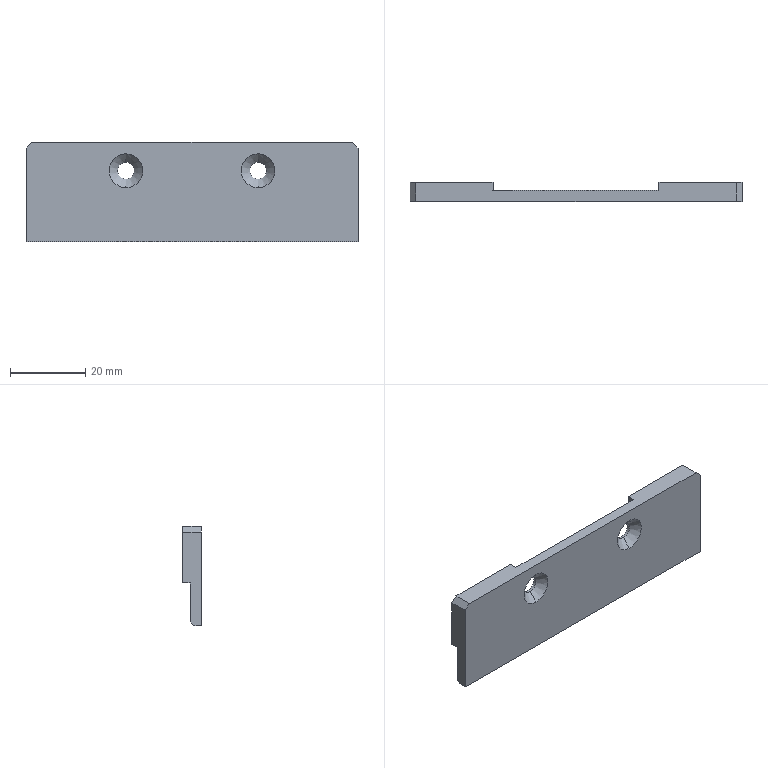Component | SolidWorks | 12-DividingMechanism-1111-1_17-1111-2 | 1 solid | 23 faces | box 88 x 5 x 26.3 mm | volume 8019 mm3 | plane 15 | cone 4 | cylinder 4 | commonest cylinder face diameters 4.5 x4
build123d program:
from build123d import *

# Parameters (mm, degrees)
SKETCH5_W                                            = 88
SKETCH5_H                                            = 26.3
BOSS_EXTRUDE1_DEPTH                                  = 5
SKETCH6_W                                            = 44
SKETCH6_H                                            = 26.3
CUT_EXTRUDE1_DEPTH                                   = 2
SKETCH7_W                                            = 88
SKETCH7_H                                            = 11.3
CUT_EXTRUDE2_DEPTH                                   = 2
CHAMFER1_SIZE                                        = 1
CHAMFER2_SIZE                                        = 1.5
M4_HEXAGON_SOCKET_COUNTERSUNK_HEAD_SCREW_D           = 4.5
M4_HEXAGON_SOCKET_COUNTERSUNK_HEAD_SCREW_CSINK_D     = 8.96
M4_HEXAGON_SOCKET_COUNTERSUNK_HEAD_SCREW_CSINK_ANGLE = 90


with BuildPart() as part:
    # Sketch5 → Boss-Extrude1 (new body)
    with BuildSketch(Plane(origin=(0, 0, 0), x_dir=(1, 0, 0), z_dir=(0, 1, 0))):
        Rectangle(SKETCH5_W, SKETCH5_H)
    extrude(amount=BOSS_EXTRUDE1_DEPTH)

    # Sketch6 → Cut-Extrude1 (cut)
    with BuildSketch(Plane(origin=(0, 5, 0), x_dir=(1, 0, 0), z_dir=(0, 1, 0))):
        Rectangle(SKETCH6_W, SKETCH6_H)
    extrude(amount=-CUT_EXTRUDE1_DEPTH, mode=Mode.SUBTRACT)

    # Sketch7 → Cut-Extrude2 (cut)
    with BuildSketch(Plane(origin=(0, 5, 0), x_dir=(1, 0, 0), z_dir=(0, 1, 0))):
        with Locations((0, -7.5)):
            Rectangle(SKETCH7_W, SKETCH7_H)
    extrude(amount=-CUT_EXTRUDE2_DEPTH, mode=Mode.SUBTRACT)

    # Chamfer1
    chamfer1_edges = [part.edges().sort_by_distance(p)[0] for p in [
        (0, 3, 13.15),
    ]]
    chamfer(chamfer1_edges, length=CHAMFER1_SIZE)

    # Chamfer2
    chamfer2_edges = [part.edges().sort_by_distance(p)[0] for p in [
        (-44, 2.5, -13.15),
        (44, 2.5, -13.15),
    ]]
    chamfer(chamfer2_edges, length=CHAMFER2_SIZE)

    # M4 Hexagon Socket Countersunk Head Screw (through all)
    with Locations(Plane(origin=(0, 0, 0), x_dir=(-1, 0, 0), z_dir=(0, -1, 0))):
        with Locations((-17.5, 5.65), (17.5, 5.65)):
            CounterSinkHole(M4_HEXAGON_SOCKET_COUNTERSUNK_HEAD_SCREW_D / 2, M4_HEXAGON_SOCKET_COUNTERSUNK_HEAD_SCREW_CSINK_D / 2, counter_sink_angle=M4_HEXAGON_SOCKET_COUNTERSUNK_HEAD_SCREW_CSINK_ANGLE)


solid = part.part

# Placed as in the assembly
solid = solid.moved(Location((3.428, 571.024, 1511.906), (-180, 0, 180)))
STEP:
#1=COLOUR_RGB('',0.7922,0.8196,0.9333);
#2=FILL_AREA_STYLE_COLOUR('',#1);
#3=FILL_AREA_STYLE('',(#2));
#4=SURFACE_STYLE_FILL_AREA(#3);
#5=SURFACE_SIDE_STYLE('',(#4));
#6=SURFACE_STYLE_USAGE(.BOTH.,#5);
#7=PRESENTATION_STYLE_ASSIGNMENT((#6));
#8=CARTESIAN_POINT('',(-0.554,22.569,59.658));
#9=VERTEX_POINT('',#8);
#10=CARTESIAN_POINT('',(-0.554,22.569,59.835));
#11=VERTEX_POINT('',#10);
#12=CARTESIAN_POINT('',(-0.554,22.569,59.746));
#13=DIRECTION('',(-0.,-1.,0.));
#14=DIRECTION('',(0.,0.,1.));
#15=AXIS2_PLACEMENT_3D('',#12,#13,#14);
#16=CIRCLE('',#15,0.08858);
#17=EDGE_CURVE('',#9,#11,#16,.T.);
#18=ORIENTED_EDGE('',*,*,#17,.F.);
#19=CARTESIAN_POINT('',(-0.554,22.481,59.57));
#20=VERTEX_POINT('',#19);
#21=CARTESIAN_POINT('',(-0.554,22.481,59.57));
#22=DIRECTION('',(-0.,-0.7071,-0.7071));
#23=VECTOR('',#22,39.37);
#24=LINE('',#21,#23);
#25=EDGE_CURVE('',#9,#20,#24,.T.);
#26=ORIENTED_EDGE('',*,*,#25,.T.);
#27=CARTESIAN_POINT('',(-0.554,22.481,59.923));
#28=VERTEX_POINT('',#27);
#29=CARTESIAN_POINT('',(-0.554,22.481,59.746));
#30=DIRECTION('',(-0.,-1.,0.));
#31=DIRECTION('',(0.,0.,1.));
#32=AXIS2_PLACEMENT_3D('',#29,#30,#31);
#33=CIRCLE('',#32,0.1764);
#34=EDGE_CURVE('',#20,#28,#33,.T.);
#35=ORIENTED_EDGE('',*,*,#34,.T.);
#36=CARTESIAN_POINT('',(-0.554,22.481,59.923));
#37=DIRECTION('',(-0.,-0.7071,0.7071));
#38=VECTOR('',#37,39.37);
#39=LINE('',#36,#38);
#40=EDGE_CURVE('',#11,#28,#39,.T.);
#41=ORIENTED_EDGE('',*,*,#40,.F.);
#42=EDGE_LOOP('',(#18,#26,#35,#41));
#43=FACE_OUTER_BOUND('',#42,.T.);
#44=CARTESIAN_POINT('',(-0.554,22.481,59.746));
#45=DIRECTION('',(-0.,-1.,0.));
#46=DIRECTION('',(0.,0.,1.));
#47=AXIS2_PLACEMENT_3D('',#44,#45,#46);
#48=CONICAL_SURFACE('',#47,0.1764,0.7854);
#49=ADVANCED_FACE('',(#43),#48,.F.);
#50=CARTESIAN_POINT('',(-0.554,22.599,59.658));
#51=VERTEX_POINT('',#50);
#52=CARTESIAN_POINT('',(-0.554,22.599,59.835));
#53=VERTEX_POINT('',#52);
#54=CARTESIAN_POINT('',(-0.554,22.599,59.746));
#55=DIRECTION('',(-0.,-1.,0.));
#56=DIRECTION('',(0.,0.,1.));
#57=AXIS2_PLACEMENT_3D('',#54,#55,#56);
#58=CIRCLE('',#57,0.08858);
#59=EDGE_CURVE('',#51,#53,#58,.T.);
#60=ORIENTED_EDGE('',*,*,#59,.F.);
#61=CARTESIAN_POINT('',(-0.554,22.481,59.658));
#62=DIRECTION('',(-0.,-1.,0.));
#63=VECTOR('',#62,39.37);
#64=LINE('',#61,#63);
#65=EDGE_CURVE('',#51,#9,#64,.T.);
#66=ORIENTED_EDGE('',*,*,#65,.T.);
#67=ORIENTED_EDGE('',*,*,#17,.T.);
#68=CARTESIAN_POINT('',(-0.554,22.481,59.835));
#69=DIRECTION('',(-0.,-1.,0.));
#70=VECTOR('',#69,39.37);
#71=LINE('',#68,#70);
#72=EDGE_CURVE('',#53,#11,#71,.T.);
#73=ORIENTED_EDGE('',*,*,#72,.F.);
#74=EDGE_LOOP('',(#60,#66,#67,#73));
#75=FACE_OUTER_BOUND('',#74,.T.);
#76=CARTESIAN_POINT('',(-0.554,22.481,59.746));
#77=DIRECTION('',(-0.,-1.,0.));
#78=DIRECTION('',(0.,0.,1.));
#79=AXIS2_PLACEMENT_3D('',#76,#77,#78);
#80=CYLINDRICAL_SURFACE('',#79,0.08858);
#81=ADVANCED_FACE('',(#75),#80,.F.);
#82=CARTESIAN_POINT('',(0.8239,22.569,59.658));
#83=VERTEX_POINT('',#82);
#84=CARTESIAN_POINT('',(0.8239,22.569,59.835));
#85=VERTEX_POINT('',#84);
#86=CARTESIAN_POINT('',(0.8239,22.569,59.746));
#87=DIRECTION('',(-0.,-1.,0.));
#88=DIRECTION('',(0.,0.,1.));
#89=AXIS2_PLACEMENT_3D('',#86,#87,#88);
#90=CIRCLE('',#89,0.08858);
#91=EDGE_CURVE('',#83,#85,#90,.T.);
#92=ORIENTED_EDGE('',*,*,#91,.F.);
#93=CARTESIAN_POINT('',(0.8239,22.481,59.57));
#94=VERTEX_POINT('',#93);
#95=CARTESIAN_POINT('',(0.8239,22.481,59.57));
#96=DIRECTION('',(-0.,-0.7071,-0.7071));
#97=VECTOR('',#96,39.37);
#98=LINE('',#95,#97);
#99=EDGE_CURVE('',#83,#94,#98,.T.);
#100=ORIENTED_EDGE('',*,*,#99,.T.);
#101=CARTESIAN_POINT('',(0.8239,22.481,59.923));
#102=VERTEX_POINT('',#101);
#103=CARTESIAN_POINT('',(0.8239,22.481,59.746));
#104=DIRECTION('',(-0.,-1.,0.));
#105=DIRECTION('',(0.,0.,1.));
#106=AXIS2_PLACEMENT_3D('',#103,#104,#105);
#107=CIRCLE('',#106,0.1764);
#108=EDGE_CURVE('',#94,#102,#107,.T.);
#109=ORIENTED_EDGE('',*,*,#108,.T.);
#110=CARTESIAN_POINT('',(0.8239,22.481,59.923));
#111=DIRECTION('',(-0.,-0.7071,0.7071));
#112=VECTOR('',#111,39.37);
#113=LINE('',#110,#112);
#114=EDGE_CURVE('',#85,#102,#113,.T.);
#115=ORIENTED_EDGE('',*,*,#114,.F.);
#116=EDGE_LOOP('',(#92,#100,#109,#115));
#117=FACE_OUTER_BOUND('',#116,.T.);
#118=CARTESIAN_POINT('',(0.8239,22.481,59.746));
#119=DIRECTION('',(-0.,-1.,0.));
#120=DIRECTION('',(0.,0.,1.));
#121=AXIS2_PLACEMENT_3D('',#118,#119,#120);
#122=CONICAL_SURFACE('',#121,0.1764,0.7854);
#123=ADVANCED_FACE('',(#117),#122,.F.);
#124=CARTESIAN_POINT('',(0.8239,22.599,59.658));
#125=VERTEX_POINT('',#124);
#126=CARTESIAN_POINT('',(0.8239,22.599,59.835));
#127=VERTEX_POINT('',#126);
#128=CARTESIAN_POINT('',(0.8239,22.599,59.746));
#129=DIRECTION('',(-0.,-1.,0.));
#130=DIRECTION('',(0.,0.,1.));
#131=AXIS2_PLACEMENT_3D('',#128,#129,#130);
#132=CIRCLE('',#131,0.08858);
#133=EDGE_CURVE('',#125,#127,#132,.T.);
#134=ORIENTED_EDGE('',*,*,#133,.F.);
#135=CARTESIAN_POINT('',(0.8239,22.481,59.658));
#136=DIRECTION('',(-0.,-1.,0.));
#137=VECTOR('',#136,39.37);
#138=LINE('',#135,#137);
#139=EDGE_CURVE('',#125,#83,#138,.T.);
#140=ORIENTED_EDGE('',*,*,#139,.T.);
#141=ORIENTED_EDGE('',*,*,#91,.T.);
#142=CARTESIAN_POINT('',(0.8239,22.481,59.835));
#143=DIRECTION('',(-0.,-1.,0.));
#144=VECTOR('',#143,39.37);
#145=LINE('',#142,#144);
#146=EDGE_CURVE('',#127,#85,#145,.T.);
#147=ORIENTED_EDGE('',*,*,#146,.F.);
#148=EDGE_LOOP('',(#134,#140,#141,#147));
#149=FACE_OUTER_BOUND('',#148,.T.);
#150=CARTESIAN_POINT('',(0.8239,22.481,59.746));
#151=DIRECTION('',(-0.,-1.,0.));
#152=DIRECTION('',(0.,0.,1.));
#153=AXIS2_PLACEMENT_3D('',#150,#151,#152);
#154=CYLINDRICAL_SURFACE('',#153,0.08858);
#155=ADVANCED_FACE('',(#149),#154,.F.);
#156=CARTESIAN_POINT('',(-1.597,22.678,59.451));
#157=VERTEX_POINT('',#156);
#158=CARTESIAN_POINT('',(-1.597,22.678,59.983));
#159=VERTEX_POINT('',#158);
#160=CARTESIAN_POINT('',(-1.597,22.678,59.006));
#161=DIRECTION('',(-0.,0.,1.));
#162=VECTOR('',#161,39.37);
#163=LINE('',#160,#162);
#164=EDGE_CURVE('',#157,#159,#163,.T.);
#165=ORIENTED_EDGE('',*,*,#164,.T.);
#166=CARTESIAN_POINT('',(-1.538,22.678,60.042));
#167=VERTEX_POINT('',#166);
#168=CARTESIAN_POINT('',(-0.9605,22.678,60.619));
#169=DIRECTION('',(0.7071,0.,0.7071));
#170=VECTOR('',#169,39.37);
#171=LINE('',#168,#170);
#172=EDGE_CURVE('',#159,#167,#171,.T.);
#173=ORIENTED_EDGE('',*,*,#172,.T.);
#174=CARTESIAN_POINT('',(-0.7312,22.678,60.042));
#175=VERTEX_POINT('',#174);
#176=CARTESIAN_POINT('',(-1.597,22.678,60.042));
#177=DIRECTION('',(1.,-0.,-0.));
#178=VECTOR('',#177,39.37);
#179=LINE('',#176,#178);
#180=EDGE_CURVE('',#167,#175,#179,.T.);
#181=ORIENTED_EDGE('',*,*,#180,.T.);
#182=CARTESIAN_POINT('',(-0.7312,22.678,59.451));
#183=VERTEX_POINT('',#182);
#184=CARTESIAN_POINT('',(-0.7312,22.678,59.006));
#185=DIRECTION('',(-0.,0.,1.));
#186=VECTOR('',#185,39.37);
#187=LINE('',#184,#186);
#188=EDGE_CURVE('',#183,#175,#187,.T.);
#189=ORIENTED_EDGE('',*,*,#188,.F.);
#190=CARTESIAN_POINT('',(1.867,22.678,59.451));
#191=DIRECTION('',(1.,-0.,0.));
#192=VECTOR('',#191,39.37);
#193=LINE('',#190,#192);
#194=EDGE_CURVE('',#157,#183,#193,.T.);
#195=ORIENTED_EDGE('',*,*,#194,.F.);
#196=EDGE_LOOP('',(#165,#173,#181,#189,#195));
#197=FACE_OUTER_BOUND('',#196,.T.);
#198=CARTESIAN_POINT('',(0.135,22.678,59.524));
#199=DIRECTION('',(0.,1.,-0.));
#200=DIRECTION('',(0.,-0.,-1.));
#201=AXIS2_PLACEMENT_3D('',#198,#199,#200);
#202=PLANE('',#201);
#203=ADVANCED_FACE('',(#197),#202,.T.);
#204=CARTESIAN_POINT('',(1.867,22.678,59.983));
#205=VERTEX_POINT('',#204);
#206=CARTESIAN_POINT('',(1.867,22.678,59.451));
#207=VERTEX_POINT('',#206);
#208=CARTESIAN_POINT('',(1.867,22.678,59.006));
#209=DIRECTION('',(0.,-0.,-1.));
#210=VECTOR('',#209,39.37);
#211=LINE('',#208,#210);
#212=EDGE_CURVE('',#205,#207,#211,.T.);
#213=ORIENTED_EDGE('',*,*,#212,.F.);
#214=CARTESIAN_POINT('',(1.867,22.481,59.983));
#215=VERTEX_POINT('',#214);
#216=CARTESIAN_POINT('',(1.867,22.678,59.983));
#217=DIRECTION('',(-0.,-1.,0.));
#218=VECTOR('',#217,39.37);
#219=LINE('',#216,#218);
#220=EDGE_CURVE('',#205,#215,#219,.T.);
#221=ORIENTED_EDGE('',*,*,#220,.T.);
#222=CARTESIAN_POINT('',(1.867,22.481,59.006));
#223=VERTEX_POINT('',#222);
#224=CARTESIAN_POINT('',(1.867,22.481,59.006));
#225=DIRECTION('',(0.,-0.,-1.));
#226=VECTOR('',#225,39.37);
#227=LINE('',#224,#226);
#228=EDGE_CURVE('',#215,#223,#227,.T.);
#229=ORIENTED_EDGE('',*,*,#228,.T.);
#230=CARTESIAN_POINT('',(1.867,22.56,59.006));
#231=VERTEX_POINT('',#230);
#232=CARTESIAN_POINT('',(1.867,22.678,59.006));
#233=DIRECTION('',(-0.,-1.,0.));
#234=VECTOR('',#233,39.37);
#235=LINE('',#232,#234);
#236=EDGE_CURVE('',#231,#223,#235,.T.);
#237=ORIENTED_EDGE('',*,*,#236,.F.);
#238=CARTESIAN_POINT('',(1.867,22.599,59.045));
#239=VERTEX_POINT('',#238);
#240=CARTESIAN_POINT('',(1.867,22.599,59.045));
#241=DIRECTION('',(0.,0.7071,0.7071));
#242=VECTOR('',#241,39.37);
#243=LINE('',#240,#242);
#244=EDGE_CURVE('',#231,#239,#243,.T.);
#245=ORIENTED_EDGE('',*,*,#244,.T.);
#246=CARTESIAN_POINT('',(1.867,22.599,59.451));
#247=VERTEX_POINT('',#246);
#248=CARTESIAN_POINT('',(1.867,22.599,59.006));
#249=DIRECTION('',(-0.,-0.,-1.));
#250=VECTOR('',#249,39.37);
#251=LINE('',#248,#250);
#252=EDGE_CURVE('',#247,#239,#251,.T.);
#253=ORIENTED_EDGE('',*,*,#252,.F.);
#254=CARTESIAN_POINT('',(1.867,22.599,59.451));
#255=DIRECTION('',(0.,1.,-0.));
#256=VECTOR('',#255,39.37);
#257=LINE('',#254,#256);
#258=EDGE_CURVE('',#247,#207,#257,.T.);
#259=ORIENTED_EDGE('',*,*,#258,.T.);
#260=EDGE_LOOP('',(#213,#221,#229,#237,#245,#253,#259));
#261=FACE_OUTER_BOUND('',#260,.T.);
#262=CARTESIAN_POINT('',(1.867,22.678,59.006));
#263=DIRECTION('',(-1.,0.,-0.));
#264=DIRECTION('',(-0.,0.,1.));
#265=AXIS2_PLACEMENT_3D('',#262,#263,#264);
#266=PLANE('',#265);
#267=ADVANCED_FACE('',(#261),#266,.F.);
#268=CARTESIAN_POINT('',(-1.597,22.56,59.006));
#269=VERTEX_POINT('',#268);
#270=CARTESIAN_POINT('',(-1.597,22.481,59.006));
#271=VERTEX_POINT('',#270);
#272=CARTESIAN_POINT('',(-1.597,22.678,59.006));
#273=DIRECTION('',(-0.,-1.,0.));
#274=VECTOR('',#273,39.37);
#275=LINE('',#272,#274);
#276=EDGE_CURVE('',#269,#271,#275,.T.);
#277=ORIENTED_EDGE('',*,*,#276,.F.);
#278=CARTESIAN_POINT('',(-1.597,22.56,59.006));
#279=DIRECTION('',(1.,-0.,-0.));
#280=VECTOR('',#279,39.37);
#281=LINE('',#278,#280);
#282=EDGE_CURVE('',#269,#231,#281,.T.);
#283=ORIENTED_EDGE('',*,*,#282,.T.);
#284=ORIENTED_EDGE('',*,*,#236,.T.);
#285=CARTESIAN_POINT('',(-1.597,22.481,59.006));
#286=DIRECTION('',(-1.,0.,0.));
#287=VECTOR('',#286,39.37);
#288=LINE('',#285,#287);
#289=EDGE_CURVE('',#223,#271,#288,.T.);
#290=ORIENTED_EDGE('',*,*,#289,.T.);
#291=EDGE_LOOP('',(#277,#283,#284,#290));
#292=FACE_OUTER_BOUND('',#291,.T.);
#293=CARTESIAN_POINT('',(-1.597,22.678,59.006));
#294=DIRECTION('',(0.,0.,1.));
#295=DIRECTION('',(1.,-0.,-0.));
#296=AXIS2_PLACEMENT_3D('',#293,#294,#295);
#297=PLANE('',#296);
#298=ADVANCED_FACE('',(#292),#297,.F.);
#299=CARTESIAN_POINT('',(-1.597,22.481,59.983));
#300=VERTEX_POINT('',#299);
#301=CARTESIAN_POINT('',(-1.597,22.481,59.006));
#302=DIRECTION('',(-0.,0.,1.));
#303=VECTOR('',#302,39.37);
#304=LINE('',#301,#303);
#305=EDGE_CURVE('',#271,#300,#304,.T.);
#306=ORIENTED_EDGE('',*,*,#305,.T.);
#307=CARTESIAN_POINT('',(-1.597,22.678,59.983));
#308=DIRECTION('',(0.,1.,-0.));
#309=VECTOR('',#308,39.37);
#310=LINE('',#307,#309);
#311=EDGE_CURVE('',#300,#159,#310,.T.);
#312=ORIENTED_EDGE('',*,*,#311,.T.);
#313=ORIENTED_EDGE('',*,*,#164,.F.);
#314=CARTESIAN_POINT('',(-1.597,22.599,59.451));
#315=VERTEX_POINT('',#314);
#316=CARTESIAN_POINT('',(-1.597,22.599,59.451));
#317=DIRECTION('',(0.,1.,-0.));
#318=VECTOR('',#317,39.37);
#319=LINE('',#316,#318);
#320=EDGE_CURVE('',#315,#157,#319,.T.);
#321=ORIENTED_EDGE('',*,*,#320,.F.);
#322=CARTESIAN_POINT('',(-1.597,22.599,59.045));
#323=VERTEX_POINT('',#322);
#324=CARTESIAN_POINT('',(-1.597,22.599,59.006));
#325=DIRECTION('',(-0.,0.,1.));
#326=VECTOR('',#325,39.37);
#327=LINE('',#324,#326);
#328=EDGE_CURVE('',#323,#315,#327,.T.);
#329=ORIENTED_EDGE('',*,*,#328,.F.);
#330=CARTESIAN_POINT('',(-1.597,22.599,59.045));
#331=DIRECTION('',(-0.,-0.7071,-0.7071));
#332=VECTOR('',#331,39.37);
#333=LINE('',#330,#332);
#334=EDGE_CURVE('',#323,#269,#333,.T.);
#335=ORIENTED_EDGE('',*,*,#334,.T.);
#336=ORIENTED_EDGE('',*,*,#276,.T.);
#337=EDGE_LOOP('',(#306,#312,#313,#321,#329,#335,#336));
#338=FACE_OUTER_BOUND('',#337,.T.);
#339=CARTESIAN_POINT('',(-1.597,22.678,59.006));
#340=DIRECTION('',(1.,-0.,0.));
#341=DIRECTION('',(0.,-0.,-1.));
#342=AXIS2_PLACEMENT_3D('',#339,#340,#341);
#343=PLANE('',#342);
#344=ADVANCED_FACE('',(#338),#343,.F.);
#345=CARTESIAN_POINT('',(-1.538,22.481,60.042));
#346=VERTEX_POINT('',#345);
#347=CARTESIAN_POINT('',(1.808,22.481,60.042));
#348=VERTEX_POINT('',#347);
#349=CARTESIAN_POINT('',(-1.597,22.481,60.042));
#350=DIRECTION('',(1.,-0.,-0.));
#351=VECTOR('',#350,39.37);
#352=LINE('',#349,#351);
#353=EDGE_CURVE('',#346,#348,#352,.T.);
#354=ORIENTED_EDGE('',*,*,#353,.T.);
#355=CARTESIAN_POINT('',(1.808,22.678,60.042));
#356=VERTEX_POINT('',#355);
#357=CARTESIAN_POINT('',(1.808,22.678,60.042));
#358=DIRECTION('',(0.,1.,-0.));
#359=VECTOR('',#358,39.37);
#360=LINE('',#357,#359);
#361=EDGE_CURVE('',#348,#356,#360,.T.);
#362=ORIENTED_EDGE('',*,*,#361,.T.);
#363=CARTESIAN_POINT('',(1.001,22.678,60.042));
#364=VERTEX_POINT('',#363);
#365=CARTESIAN_POINT('',(-1.597,22.678,60.042));
#366=DIRECTION('',(1.,-0.,-0.));
#367=VECTOR('',#366,39.37);
#368=LINE('',#365,#367);
#369=EDGE_CURVE('',#364,#356,#368,.T.);
#370=ORIENTED_EDGE('',*,*,#369,.F.);
#371=CARTESIAN_POINT('',(1.001,22.599,60.042));
#372=VERTEX_POINT('',#371);
#373=CARTESIAN_POINT('',(1.001,22.599,60.042));
#374=DIRECTION('',(0.,1.,-0.));
#375=VECTOR('',#374,39.37);
#376=LINE('',#373,#375);
#377=EDGE_CURVE('',#372,#364,#376,.T.);
#378=ORIENTED_EDGE('',*,*,#377,.F.);
#379=CARTESIAN_POINT('',(-0.7312,22.599,60.042));
#380=VERTEX_POINT('',#379);
#381=CARTESIAN_POINT('',(1.001,22.599,60.042));
#382=DIRECTION('',(1.,-0.,0.));
#383=VECTOR('',#382,39.37);
#384=LINE('',#381,#383);
#385=EDGE_CURVE('',#380,#372,#384,.T.);
#386=ORIENTED_EDGE('',*,*,#385,.F.);
#387=CARTESIAN_POINT('',(-0.7312,22.599,60.042));
#388=DIRECTION('',(0.,1.,-0.));
#389=VECTOR('',#388,39.37);
#390=LINE('',#387,#389);
#391=EDGE_CURVE('',#380,#175,#390,.T.);
#392=ORIENTED_EDGE('',*,*,#391,.T.);
#393=ORIENTED_EDGE('',*,*,#180,.F.);
#394=CARTESIAN_POINT('',(-1.538,22.678,60.042));
#395=DIRECTION('',(-0.,-1.,0.));
#396=VECTOR('',#395,39.37);
#397=LINE('',#394,#396);
#398=EDGE_CURVE('',#167,#346,#397,.T.);
#399=ORIENTED_EDGE('',*,*,#398,.T.);
#400=EDGE_LOOP('',(#354,#362,#370,#378,#386,#392,#393,#399));
#401=FACE_OUTER_BOUND('',#400,.T.);
#402=CARTESIAN_POINT('',(-1.597,22.678,60.042));
#403=DIRECTION('',(-0.,-0.,-1.));
#404=DIRECTION('',(-1.,0.,0.));
#405=AXIS2_PLACEMENT_3D('',#402,#403,#404);
#406=PLANE('',#405);
#407=ADVANCED_FACE('',(#401),#406,.F.);
#408=ORIENTED_EDGE('',*,*,#369,.T.);
#409=CARTESIAN_POINT('',(1.23,22.678,60.619));
#410=DIRECTION('',(0.7071,-0.,-0.7071));
#411=VECTOR('',#410,39.37);
#412=LINE('',#409,#411);
#413=EDGE_CURVE('',#356,#205,#412,.T.);
#414=ORIENTED_EDGE('',*,*,#413,.T.);
#415=ORIENTED_EDGE('',*,*,#212,.T.);
#416=CARTESIAN_POINT('',(1.001,22.678,59.451));
#417=VERTEX_POINT('',#416);
#418=CARTESIAN_POINT('',(1.867,22.678,59.451));
#419=DIRECTION('',(1.,-0.,0.));
#420=VECTOR('',#419,39.37);
#421=LINE('',#418,#420);
#422=EDGE_CURVE('',#417,#207,#421,.T.);
#423=ORIENTED_EDGE('',*,*,#422,.F.);
#424=CARTESIAN_POINT('',(1.001,22.678,59.006));
#425=DIRECTION('',(0.,-0.,-1.));
#426=VECTOR('',#425,39.37);
#427=LINE('',#424,#426);
#428=EDGE_CURVE('',#364,#417,#427,.T.);
#429=ORIENTED_EDGE('',*,*,#428,.F.);
#430=EDGE_LOOP('',(#408,#414,#415,#423,#429));
#431=FACE_OUTER_BOUND('',#430,.T.);
#432=CARTESIAN_POINT('',(0.135,22.678,59.524));
#433=DIRECTION('',(0.,1.,-0.));
#434=DIRECTION('',(0.,-0.,-1.));
#435=AXIS2_PLACEMENT_3D('',#432,#433,#434);
#436=PLANE('',#435);
#437=ADVANCED_FACE('',(#431),#436,.T.);
#438=CARTESIAN_POINT('',(-0.554,22.481,59.746));
#439=DIRECTION('',(-0.,-1.,0.));
#440=DIRECTION('',(0.,0.,1.));
#441=AXIS2_PLACEMENT_3D('',#438,#439,#440);
#442=CIRCLE('',#441,0.1764);
#443=EDGE_CURVE('',#28,#20,#442,.T.);
#444=ORIENTED_EDGE('',*,*,#443,.F.);
#445=ORIENTED_EDGE('',*,*,#34,.F.);
#446=EDGE_LOOP('',(#444,#445));
#447=FACE_BOUND('',#446,.T.);
#448=CARTESIAN_POINT('',(0.8239,22.481,59.746));
#449=DIRECTION('',(-0.,-1.,0.));
#450=DIRECTION('',(0.,0.,1.));
#451=AXIS2_PLACEMENT_3D('',#448,#449,#450);
#452=CIRCLE('',#451,0.1764);
#453=EDGE_CURVE('',#102,#94,#452,.T.);
#454=ORIENTED_EDGE('',*,*,#453,.F.);
#455=ORIENTED_EDGE('',*,*,#108,.F.);
#456=EDGE_LOOP('',(#454,#455));
#457=FACE_BOUND('',#456,.T.);
#458=ORIENTED_EDGE('',*,*,#228,.F.);
#459=CARTESIAN_POINT('',(1.867,22.481,59.983));
#460=DIRECTION('',(-0.7071,0.,0.7071));
#461=VECTOR('',#460,39.37);
#462=LINE('',#459,#461);
#463=EDGE_CURVE('',#215,#348,#462,.T.);
#464=ORIENTED_EDGE('',*,*,#463,.T.);
#465=ORIENTED_EDGE('',*,*,#353,.F.);
#466=CARTESIAN_POINT('',(-1.538,22.481,60.042));
#467=DIRECTION('',(-0.7071,-0.,-0.7071));
#468=VECTOR('',#467,39.37);
#469=LINE('',#466,#468);
#470=EDGE_CURVE('',#346,#300,#469,.T.);
#471=ORIENTED_EDGE('',*,*,#470,.T.);
#472=ORIENTED_EDGE('',*,*,#305,.F.);
#473=ORIENTED_EDGE('',*,*,#289,.F.);
#474=EDGE_LOOP('',(#458,#464,#465,#471,#472,#473));
#475=FACE_OUTER_BOUND('',#474,.T.);
#476=CARTESIAN_POINT('',(0.135,22.481,59.524));
#477=DIRECTION('',(0.,1.,-0.));
#478=DIRECTION('',(0.,-0.,-1.));
#479=AXIS2_PLACEMENT_3D('',#476,#477,#478);
#480=PLANE('',#479);
#481=ADVANCED_FACE('',(#447,#457,#475),#480,.F.);
#482=CARTESIAN_POINT('',(-0.7312,22.599,59.451));
#483=VERTEX_POINT('',#482);
#484=CARTESIAN_POINT('',(-0.7312,22.599,59.006));
#485=DIRECTION('',(-0.,0.,1.));
#486=VECTOR('',#485,39.37);
#487=LINE('',#484,#486);
#488=EDGE_CURVE('',#483,#380,#487,.T.);
#489=ORIENTED_EDGE('',*,*,#488,.F.);
#490=CARTESIAN_POINT('',(-0.7312,22.599,59.451));
#491=DIRECTION('',(0.,1.,-0.));
#492=VECTOR('',#491,39.37);
#493=LINE('',#490,#492);
#494=EDGE_CURVE('',#483,#183,#493,.T.);
#495=ORIENTED_EDGE('',*,*,#494,.T.);
#496=ORIENTED_EDGE('',*,*,#188,.T.);
#497=ORIENTED_EDGE('',*,*,#391,.F.);
#498=EDGE_LOOP('',(#489,#495,#496,#497));
#499=FACE_OUTER_BOUND('',#498,.T.);
#500=CARTESIAN_POINT('',(-0.7312,22.599,59.006));
#501=DIRECTION('',(-1.,0.,-0.));
#502=DIRECTION('',(-0.,0.,1.));
#503=AXIS2_PLACEMENT_3D('',#500,#501,#502);
#504=PLANE('',#503);
#505=ADVANCED_FACE('',(#499),#504,.F.);
#506=ORIENTED_EDGE('',*,*,#428,.T.);
#507=CARTESIAN_POINT('',(1.001,22.599,59.451));
#508=VERTEX_POINT('',#507);
#509=CARTESIAN_POINT('',(1.001,22.599,59.451));
#510=DIRECTION('',(-0.,-1.,0.));
#511=VECTOR('',#510,39.37);
#512=LINE('',#509,#511);
#513=EDGE_CURVE('',#417,#508,#512,.T.);
#514=ORIENTED_EDGE('',*,*,#513,.T.);
#515=CARTESIAN_POINT('',(1.001,22.599,59.006));
#516=DIRECTION('',(0.,-0.,-1.));
#517=VECTOR('',#516,39.37);
#518=LINE('',#515,#517);
#519=EDGE_CURVE('',#372,#508,#518,.T.);
#520=ORIENTED_EDGE('',*,*,#519,.F.);
#521=ORIENTED_EDGE('',*,*,#377,.T.);
#522=EDGE_LOOP('',(#506,#514,#520,#521));
#523=FACE_OUTER_BOUND('',#522,.T.);
#524=CARTESIAN_POINT('',(1.001,22.599,59.006));
#525=DIRECTION('',(1.,-0.,0.));
#526=DIRECTION('',(0.,-0.,-1.));
#527=AXIS2_PLACEMENT_3D('',#524,#525,#526);
#528=PLANE('',#527);
#529=ADVANCED_FACE('',(#523),#528,.F.);
#530=CARTESIAN_POINT('',(-0.554,22.599,59.746));
#531=DIRECTION('',(-0.,-1.,0.));
#532=DIRECTION('',(0.,0.,1.));
#533=AXIS2_PLACEMENT_3D('',#530,#531,#532);
#534=CIRCLE('',#533,0.08858);
#535=EDGE_CURVE('',#53,#51,#534,.T.);
#536=ORIENTED_EDGE('',*,*,#535,.T.);
#537=ORIENTED_EDGE('',*,*,#59,.T.);
#538=EDGE_LOOP('',(#536,#537));
#539=FACE_BOUND('',#538,.T.);
#540=CARTESIAN_POINT('',(0.8239,22.599,59.746));
#541=DIRECTION('',(-0.,-1.,0.));
#542=DIRECTION('',(0.,0.,1.));
#543=AXIS2_PLACEMENT_3D('',#540,#541,#542);
#544=CIRCLE('',#543,0.08858);
#545=EDGE_CURVE('',#127,#125,#544,.T.);
#546=ORIENTED_EDGE('',*,*,#545,.T.);
#547=ORIENTED_EDGE('',*,*,#133,.T.);
#548=EDGE_LOOP('',(#546,#547));
#549=FACE_BOUND('',#548,.T.);
#550=ORIENTED_EDGE('',*,*,#252,.T.);
#551=CARTESIAN_POINT('',(0.135,22.599,59.045));
#552=DIRECTION('',(-1.,0.,0.));
#553=VECTOR('',#552,39.37);
#554=LINE('',#551,#553);
#555=EDGE_CURVE('',#239,#323,#554,.T.);
#556=ORIENTED_EDGE('',*,*,#555,.T.);
#557=ORIENTED_EDGE('',*,*,#328,.T.);
#558=CARTESIAN_POINT('',(1.867,22.599,59.451));
#559=DIRECTION('',(1.,-0.,0.));
#560=VECTOR('',#559,39.37);
#561=LINE('',#558,#560);
#562=EDGE_CURVE('',#315,#483,#561,.T.);
#563=ORIENTED_EDGE('',*,*,#562,.T.);
#564=ORIENTED_EDGE('',*,*,#488,.T.);
#565=ORIENTED_EDGE('',*,*,#385,.T.);
#566=ORIENTED_EDGE('',*,*,#519,.T.);
#567=CARTESIAN_POINT('',(1.867,22.599,59.451));
#568=DIRECTION('',(1.,-0.,0.));
#569=VECTOR('',#568,39.37);
#570=LINE('',#567,#569);
#571=EDGE_CURVE('',#508,#247,#570,.T.);
#572=ORIENTED_EDGE('',*,*,#571,.T.);
#573=EDGE_LOOP('',(#550,#556,#557,#563,#564,#565,#566,#572));
#574=FACE_OUTER_BOUND('',#573,.T.);
#575=CARTESIAN_POINT('',(0.135,22.599,59.524));
#576=DIRECTION('',(-0.,-1.,0.));
#577=DIRECTION('',(-0.,0.,1.));
#578=AXIS2_PLACEMENT_3D('',#575,#576,#577);
#579=PLANE('',#578);
#580=ADVANCED_FACE('',(#539,#549,#574),#579,.F.);
#581=ORIENTED_EDGE('',*,*,#422,.T.);
#582=ORIENTED_EDGE('',*,*,#258,.F.);
#583=ORIENTED_EDGE('',*,*,#571,.F.);
#584=ORIENTED_EDGE('',*,*,#513,.F.);
#585=EDGE_LOOP('',(#581,#582,#583,#584));
#586=FACE_OUTER_BOUND('',#585,.T.);
#587=CARTESIAN_POINT('',(1.867,22.599,59.451));
#588=DIRECTION('',(-0.,0.,1.));
#589=DIRECTION('',(1.,-0.,0.));
#590=AXIS2_PLACEMENT_3D('',#587,#588,#589);
#591=PLANE('',#590);
#592=ADVANCED_FACE('',(#586),#591,.F.);
#593=ORIENTED_EDGE('',*,*,#562,.F.);
#594=ORIENTED_EDGE('',*,*,#320,.T.);
#595=ORIENTED_EDGE('',*,*,#194,.T.);
#596=ORIENTED_EDGE('',*,*,#494,.F.);
#597=EDGE_LOOP('',(#593,#594,#595,#596));
#598=FACE_OUTER_BOUND('',#597,.T.);
#599=CARTESIAN_POINT('',(1.867,22.599,59.451));
#600=DIRECTION('',(-0.,0.,1.));
#601=DIRECTION('',(1.,-0.,0.));
#602=AXIS2_PLACEMENT_3D('',#599,#600,#601);
#603=PLANE('',#602);
#604=ADVANCED_FACE('',(#598),#603,.F.);
#605=ORIENTED_EDGE('',*,*,#244,.F.);
#606=ORIENTED_EDGE('',*,*,#282,.F.);
#607=ORIENTED_EDGE('',*,*,#334,.F.);
#608=ORIENTED_EDGE('',*,*,#555,.F.);
#609=EDGE_LOOP('',(#605,#606,#607,#608));
#610=FACE_OUTER_BOUND('',#609,.T.);
#611=CARTESIAN_POINT('',(0.135,22.599,59.045));
#612=DIRECTION('',(0.,-0.7071,0.7071));
#613=DIRECTION('',(-1.,0.,0.));
#614=AXIS2_PLACEMENT_3D('',#611,#612,#613);
#615=PLANE('',#614);
#616=ADVANCED_FACE('',(#610),#615,.F.);
#617=ORIENTED_EDGE('',*,*,#413,.F.);
#618=ORIENTED_EDGE('',*,*,#361,.F.);
#619=ORIENTED_EDGE('',*,*,#463,.F.);
#620=ORIENTED_EDGE('',*,*,#220,.F.);
#621=EDGE_LOOP('',(#617,#618,#619,#620));
#622=FACE_OUTER_BOUND('',#621,.T.);
#623=CARTESIAN_POINT('',(1.867,22.678,59.983));
#624=DIRECTION('',(-0.7071,-0.,-0.7071));
#625=DIRECTION('',(-0.,-1.,0.));
#626=AXIS2_PLACEMENT_3D('',#623,#624,#625);
#627=PLANE('',#626);
#628=ADVANCED_FACE('',(#622),#627,.F.);
#629=ORIENTED_EDGE('',*,*,#172,.F.);
#630=ORIENTED_EDGE('',*,*,#311,.F.);
#631=ORIENTED_EDGE('',*,*,#470,.F.);
#632=ORIENTED_EDGE('',*,*,#398,.F.);
#633=EDGE_LOOP('',(#629,#630,#631,#632));
#634=FACE_OUTER_BOUND('',#633,.T.);
#635=CARTESIAN_POINT('',(-1.538,22.678,60.042));
#636=DIRECTION('',(0.7071,-0.,-0.7071));
#637=DIRECTION('',(-0.,-1.,0.));
#638=AXIS2_PLACEMENT_3D('',#635,#636,#637);
#639=PLANE('',#638);
#640=ADVANCED_FACE('',(#634),#639,.F.);
#641=ORIENTED_EDGE('',*,*,#139,.F.);
#642=ORIENTED_EDGE('',*,*,#545,.F.);
#643=ORIENTED_EDGE('',*,*,#146,.T.);
#644=CARTESIAN_POINT('',(0.8239,22.569,59.746));
#645=DIRECTION('',(-0.,-1.,0.));
#646=DIRECTION('',(0.,0.,1.));
#647=AXIS2_PLACEMENT_3D('',#644,#645,#646);
#648=CIRCLE('',#647,0.08858);
#649=EDGE_CURVE('',#85,#83,#648,.T.);
#650=ORIENTED_EDGE('',*,*,#649,.T.);
#651=EDGE_LOOP('',(#641,#642,#643,#650));
#652=FACE_OUTER_BOUND('',#651,.T.);
#653=CARTESIAN_POINT('',(0.8239,22.481,59.746));
#654=DIRECTION('',(-0.,-1.,0.));
#655=DIRECTION('',(0.,0.,1.));
#656=AXIS2_PLACEMENT_3D('',#653,#654,#655);
#657=CYLINDRICAL_SURFACE('',#656,0.08858);
#658=ADVANCED_FACE('',(#652),#657,.F.);
#659=ORIENTED_EDGE('',*,*,#99,.F.);
#660=ORIENTED_EDGE('',*,*,#649,.F.);
#661=ORIENTED_EDGE('',*,*,#114,.T.);
#662=ORIENTED_EDGE('',*,*,#453,.T.);
#663=EDGE_LOOP('',(#659,#660,#661,#662));
#664=FACE_OUTER_BOUND('',#663,.T.);
#665=CARTESIAN_POINT('',(0.8239,22.481,59.746));
#666=DIRECTION('',(-0.,-1.,0.));
#667=DIRECTION('',(0.,0.,1.));
#668=AXIS2_PLACEMENT_3D('',#665,#666,#667);
#669=CONICAL_SURFACE('',#668,0.1764,0.7854);
#670=ADVANCED_FACE('',(#664),#669,.F.);
#671=ORIENTED_EDGE('',*,*,#65,.F.);
#672=ORIENTED_EDGE('',*,*,#535,.F.);
#673=ORIENTED_EDGE('',*,*,#72,.T.);
#674=CARTESIAN_POINT('',(-0.554,22.569,59.746));
#675=DIRECTION('',(-0.,-1.,0.));
#676=DIRECTION('',(0.,0.,1.));
#677=AXIS2_PLACEMENT_3D('',#674,#675,#676);
#678=CIRCLE('',#677,0.08858);
#679=EDGE_CURVE('',#11,#9,#678,.T.);
#680=ORIENTED_EDGE('',*,*,#679,.T.);
#681=EDGE_LOOP('',(#671,#672,#673,#680));
#682=FACE_OUTER_BOUND('',#681,.T.);
#683=CARTESIAN_POINT('',(-0.554,22.481,59.746));
#684=DIRECTION('',(-0.,-1.,0.));
#685=DIRECTION('',(0.,0.,1.));
#686=AXIS2_PLACEMENT_3D('',#683,#684,#685);
#687=CYLINDRICAL_SURFACE('',#686,0.08858);
#688=ADVANCED_FACE('',(#682),#687,.F.);
#689=ORIENTED_EDGE('',*,*,#25,.F.);
#690=ORIENTED_EDGE('',*,*,#679,.F.);
#691=ORIENTED_EDGE('',*,*,#40,.T.);
#692=ORIENTED_EDGE('',*,*,#443,.T.);
#693=EDGE_LOOP('',(#689,#690,#691,#692));
#694=FACE_OUTER_BOUND('',#693,.T.);
#695=CARTESIAN_POINT('',(-0.554,22.481,59.746));
#696=DIRECTION('',(-0.,-1.,0.));
#697=DIRECTION('',(0.,0.,1.));
#698=AXIS2_PLACEMENT_3D('',#695,#696,#697);
#699=CONICAL_SURFACE('',#698,0.1764,0.7854);
#700=ADVANCED_FACE('',(#694),#699,.F.);
#701=CLOSED_SHELL('',(#49,#81,#123,#155,#203,#267,#298,#344,#407,#437,#481,#505,#529,#580,#592,#604,#616,#628,#640,#658,#670,#688,#700));
#702=MANIFOLD_SOLID_BREP('',#701);
#703=STYLED_ITEM('',(#7),#702);
#704=(LENGTH_UNIT()NAMED_UNIT(*)SI_UNIT($,.METRE.));
#705=LENGTH_MEASURE_WITH_UNIT(LENGTH_MEASURE(0.0254),#704);
#706=DIMENSIONAL_EXPONENTS(1.,0.,0.,0.,0.,0.,0.);
#707=(CONVERSION_BASED_UNIT('',#705)LENGTH_UNIT()NAMED_UNIT(#706));
#708=UNCERTAINTY_MEASURE_WITH_UNIT(LENGTH_MEASURE(0.00001),#707,'','');
#709=(NAMED_UNIT(*)PLANE_ANGLE_UNIT()SI_UNIT($,.RADIAN.));
#710=(NAMED_UNIT(*)SI_UNIT($,.STERADIAN.)SOLID_ANGLE_UNIT());
#711=(GEOMETRIC_REPRESENTATION_CONTEXT(3)GLOBAL_UNCERTAINTY_ASSIGNED_CONTEXT((#708))GLOBAL_UNIT_ASSIGNED_CONTEXT((#707,#709,#710))REPRESENTATION_CONTEXT('',''));
#712=MECHANICAL_DESIGN_GEOMETRIC_PRESENTATION_REPRESENTATION('',(#703),#711);
#713=PRESENTATION_LAYER_ASSIGNMENT('','',(#703));
#714=CARTESIAN_POINT('',(0.,0.,0.));
#715=DIRECTION('',(0.,0.,1.));
#716=DIRECTION('',(1.,0.,0.));
#717=AXIS2_PLACEMENT_3D('',#714,#715,#716);
#718=(LENGTH_UNIT()NAMED_UNIT(*)SI_UNIT($,.METRE.));
#719=LENGTH_MEASURE_WITH_UNIT(LENGTH_MEASURE(0.0254),#718);
#720=DIMENSIONAL_EXPONENTS(1.,0.,0.,0.,0.,0.,0.);
#721=(CONVERSION_BASED_UNIT('',#719)LENGTH_UNIT()NAMED_UNIT(#720));
#722=UNCERTAINTY_MEASURE_WITH_UNIT(LENGTH_MEASURE(0.00001),#721,'','');
#723=(NAMED_UNIT(*)PLANE_ANGLE_UNIT()SI_UNIT($,.RADIAN.));
#724=(NAMED_UNIT(*)SI_UNIT($,.STERADIAN.)SOLID_ANGLE_UNIT());
#725=(GEOMETRIC_REPRESENTATION_CONTEXT(3)GLOBAL_UNCERTAINTY_ASSIGNED_CONTEXT((#722))GLOBAL_UNIT_ASSIGNED_CONTEXT((#721,#723,#724))REPRESENTATION_CONTEXT('',''));
#726=ADVANCED_BREP_SHAPE_REPRESENTATION('',(#702,#717),#725);